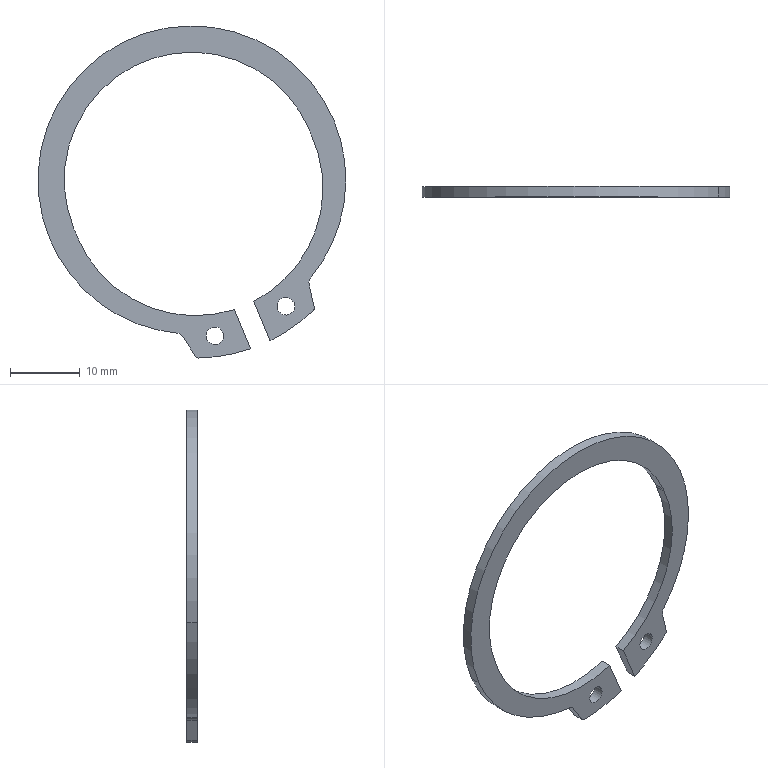Component | SolidWorks | BearingHousingAssembly-1_40ShaftRetainingRing-1 | 1 solid | 25 faces | box 44 x 1.5 x 47.45 mm | volume 704 mm3 | cylinder 19 | plane 6 | commonest cylinder face diameters 36.5 x6 2.5 x4 44 x3 2 x2 48.6 x2 1 x2
STEP:
#1=COLOUR_RGB('',0.7922,0.8196,0.9333);
#2=FILL_AREA_STYLE_COLOUR('',#1);
#3=FILL_AREA_STYLE('',(#2));
#4=SURFACE_STYLE_FILL_AREA(#3);
#5=SURFACE_SIDE_STYLE('',(#4));
#6=SURFACE_STYLE_USAGE(.BOTH.,#5);
#7=PRESENTATION_STYLE_ASSIGNMENT((#6));
#8=CARTESIAN_POINT('',(-0.8586,9.341,0.039));
#9=VERTEX_POINT('',#8);
#10=CARTESIAN_POINT('',(-0.8495,9.341,0.01611));
#11=VERTEX_POINT('',#10);
#12=CARTESIAN_POINT('',(-1.522,9.341,-0.2362));
#13=DIRECTION('',(0.,1.,0.));
#14=DIRECTION('',(-0.9237,0.,-0.383));
#15=AXIS2_PLACEMENT_3D('',#12,#13,#14);
#16=CIRCLE('',#15,0.7185);
#17=EDGE_CURVE('',#9,#11,#16,.T.);
#18=ORIENTED_EDGE('',*,*,#17,.F.);
#19=CARTESIAN_POINT('',(-0.8586,9.4,0.039));
#20=VERTEX_POINT('',#19);
#21=CARTESIAN_POINT('',(-0.8586,9.341,0.039));
#22=DIRECTION('',(0.,1.,0.));
#23=VECTOR('',#22,39.37);
#24=LINE('',#21,#23);
#25=EDGE_CURVE('',#9,#20,#24,.T.);
#26=ORIENTED_EDGE('',*,*,#25,.T.);
#27=CARTESIAN_POINT('',(-0.8495,9.4,0.01611));
#28=VERTEX_POINT('',#27);
#29=CARTESIAN_POINT('',(-1.522,9.4,-0.2362));
#30=DIRECTION('',(0.,1.,0.));
#31=DIRECTION('',(-0.9237,0.,-0.383));
#32=AXIS2_PLACEMENT_3D('',#29,#30,#31);
#33=CIRCLE('',#32,0.7185);
#34=EDGE_CURVE('',#20,#28,#33,.T.);
#35=ORIENTED_EDGE('',*,*,#34,.T.);
#36=CARTESIAN_POINT('',(-0.8495,9.371,0.01611));
#37=DIRECTION('',(0.,1.,0.));
#38=VECTOR('',#37,39.37);
#39=LINE('',#36,#38);
#40=EDGE_CURVE('',#11,#28,#39,.T.);
#41=ORIENTED_EDGE('',*,*,#40,.F.);
#42=EDGE_LOOP('',(#18,#26,#35,#41));
#43=FACE_OUTER_BOUND('',#42,.T.);
#44=CARTESIAN_POINT('',(-1.522,9.341,-0.2362));
#45=DIRECTION('',(0.,1.,0.));
#46=DIRECTION('',(-0.9237,0.,-0.383));
#47=AXIS2_PLACEMENT_3D('',#44,#45,#46);
#48=CYLINDRICAL_SURFACE('',#47,0.7185);
#49=ADVANCED_FACE('',(#43),#48,.F.);
#50=ORIENTED_EDGE('',*,*,#25,.F.);
#51=CARTESIAN_POINT('',(-2.186,9.341,-0.5114));
#52=VERTEX_POINT('',#51);
#53=CARTESIAN_POINT('',(-1.522,9.341,-0.2362));
#54=DIRECTION('',(0.,1.,0.));
#55=DIRECTION('',(-0.9237,0.,-0.383));
#56=AXIS2_PLACEMENT_3D('',#53,#54,#55);
#57=CIRCLE('',#56,0.7185);
#58=EDGE_CURVE('',#52,#9,#57,.T.);
#59=ORIENTED_EDGE('',*,*,#58,.F.);
#60=CARTESIAN_POINT('',(-2.186,9.4,-0.5114));
#61=VERTEX_POINT('',#60);
#62=CARTESIAN_POINT('',(-2.186,9.341,-0.5114));
#63=DIRECTION('',(0.,1.,0.));
#64=VECTOR('',#63,39.37);
#65=LINE('',#62,#64);
#66=EDGE_CURVE('',#52,#61,#65,.T.);
#67=ORIENTED_EDGE('',*,*,#66,.T.);
#68=CARTESIAN_POINT('',(-1.522,9.4,-0.2362));
#69=DIRECTION('',(0.,1.,0.));
#70=DIRECTION('',(-0.9237,0.,-0.383));
#71=AXIS2_PLACEMENT_3D('',#68,#69,#70);
#72=CIRCLE('',#71,0.7185);
#73=EDGE_CURVE('',#61,#20,#72,.T.);
#74=ORIENTED_EDGE('',*,*,#73,.T.);
#75=EDGE_LOOP('',(#50,#59,#67,#74));
#76=FACE_OUTER_BOUND('',#75,.T.);
#77=CARTESIAN_POINT('',(-1.522,9.341,-0.2362));
#78=DIRECTION('',(0.,1.,0.));
#79=DIRECTION('',(-0.9237,0.,-0.383));
#80=AXIS2_PLACEMENT_3D('',#77,#78,#79);
#81=CYLINDRICAL_SURFACE('',#80,0.7185);
#82=ADVANCED_FACE('',(#76),#81,.F.);
#83=CARTESIAN_POINT('',(-2.322,9.341,-0.568));
#84=VERTEX_POINT('',#83);
#85=CARTESIAN_POINT('',(-0.7222,9.341,0.09555));
#86=VERTEX_POINT('',#85);
#87=CARTESIAN_POINT('',(-1.522,9.341,-0.2362));
#88=DIRECTION('',(0.,1.,0.));
#89=DIRECTION('',(-0.9237,0.,-0.383));
#90=AXIS2_PLACEMENT_3D('',#87,#88,#89);
#91=CIRCLE('',#90,0.8661);
#92=EDGE_CURVE('',#84,#86,#91,.T.);
#93=ORIENTED_EDGE('',*,*,#92,.T.);
#94=CARTESIAN_POINT('',(-0.7222,9.4,0.09555));
#95=VERTEX_POINT('',#94);
#96=CARTESIAN_POINT('',(-0.7222,9.341,0.09555));
#97=DIRECTION('',(0.,1.,0.));
#98=VECTOR('',#97,39.37);
#99=LINE('',#96,#98);
#100=EDGE_CURVE('',#86,#95,#99,.T.);
#101=ORIENTED_EDGE('',*,*,#100,.T.);
#102=CARTESIAN_POINT('',(-2.322,9.4,-0.568));
#103=VERTEX_POINT('',#102);
#104=CARTESIAN_POINT('',(-1.522,9.4,-0.2362));
#105=DIRECTION('',(-0.,-1.,-0.));
#106=DIRECTION('',(-0.9237,0.,-0.383));
#107=AXIS2_PLACEMENT_3D('',#104,#105,#106);
#108=CIRCLE('',#107,0.8661);
#109=EDGE_CURVE('',#95,#103,#108,.T.);
#110=ORIENTED_EDGE('',*,*,#109,.T.);
#111=CARTESIAN_POINT('',(-2.322,9.341,-0.568));
#112=DIRECTION('',(0.,1.,0.));
#113=VECTOR('',#112,39.37);
#114=LINE('',#111,#113);
#115=EDGE_CURVE('',#84,#103,#114,.T.);
#116=ORIENTED_EDGE('',*,*,#115,.F.);
#117=EDGE_LOOP('',(#93,#101,#110,#116));
#118=FACE_OUTER_BOUND('',#117,.T.);
#119=CARTESIAN_POINT('',(-1.522,9.341,-0.2362));
#120=DIRECTION('',(0.,1.,0.));
#121=DIRECTION('',(-0.9237,0.,-0.383));
#122=AXIS2_PLACEMENT_3D('',#119,#120,#121);
#123=CYLINDRICAL_SURFACE('',#122,0.8661);
#124=ADVANCED_FACE('',(#118),#123,.T.);
#125=CARTESIAN_POINT('',(-1.603,9.341,-1.099));
#126=VERTEX_POINT('',#125);
#127=CARTESIAN_POINT('',(-1.522,9.341,-0.2362));
#128=DIRECTION('',(0.,1.,0.));
#129=DIRECTION('',(-0.9237,0.,-0.383));
#130=AXIS2_PLACEMENT_3D('',#127,#128,#129);
#131=CIRCLE('',#130,0.8661);
#132=EDGE_CURVE('',#126,#84,#131,.T.);
#133=ORIENTED_EDGE('',*,*,#132,.T.);
#134=ORIENTED_EDGE('',*,*,#115,.T.);
#135=CARTESIAN_POINT('',(-1.603,9.4,-1.099));
#136=VERTEX_POINT('',#135);
#137=CARTESIAN_POINT('',(-1.522,9.4,-0.2362));
#138=DIRECTION('',(-0.,-1.,-0.));
#139=DIRECTION('',(-0.9237,0.,-0.383));
#140=AXIS2_PLACEMENT_3D('',#137,#138,#139);
#141=CIRCLE('',#140,0.8661);
#142=EDGE_CURVE('',#103,#136,#141,.T.);
#143=ORIENTED_EDGE('',*,*,#142,.T.);
#144=CARTESIAN_POINT('',(-1.603,9.341,-1.099));
#145=DIRECTION('',(-0.,-1.,-0.));
#146=VECTOR('',#145,39.37);
#147=LINE('',#144,#146);
#148=EDGE_CURVE('',#136,#126,#147,.T.);
#149=ORIENTED_EDGE('',*,*,#148,.T.);
#150=EDGE_LOOP('',(#133,#134,#143,#149));
#151=FACE_OUTER_BOUND('',#150,.T.);
#152=CARTESIAN_POINT('',(-1.522,9.341,-0.2362));
#153=DIRECTION('',(0.,1.,0.));
#154=DIRECTION('',(-0.9237,0.,-0.383));
#155=AXIS2_PLACEMENT_3D('',#152,#153,#154);
#156=CYLINDRICAL_SURFACE('',#155,0.8661);
#157=ADVANCED_FACE('',(#151),#156,.T.);
#158=CARTESIAN_POINT('',(-2.167,9.341,-0.5569));
#159=VERTEX_POINT('',#158);
#160=CARTESIAN_POINT('',(-2.176,9.341,-0.534));
#161=VERTEX_POINT('',#160);
#162=CARTESIAN_POINT('',(-1.503,9.341,-0.2817));
#163=DIRECTION('',(0.,1.,0.));
#164=DIRECTION('',(-0.9237,0.,-0.383));
#165=AXIS2_PLACEMENT_3D('',#162,#163,#164);
#166=CIRCLE('',#165,0.7185);
#167=EDGE_CURVE('',#159,#161,#166,.T.);
#168=ORIENTED_EDGE('',*,*,#167,.F.);
#169=CARTESIAN_POINT('',(-2.167,9.4,-0.5569));
#170=VERTEX_POINT('',#169);
#171=CARTESIAN_POINT('',(-2.167,9.341,-0.5569));
#172=DIRECTION('',(0.,1.,0.));
#173=VECTOR('',#172,39.37);
#174=LINE('',#171,#173);
#175=EDGE_CURVE('',#159,#170,#174,.T.);
#176=ORIENTED_EDGE('',*,*,#175,.T.);
#177=CARTESIAN_POINT('',(-2.176,9.4,-0.534));
#178=VERTEX_POINT('',#177);
#179=CARTESIAN_POINT('',(-1.503,9.4,-0.2817));
#180=DIRECTION('',(0.,1.,0.));
#181=DIRECTION('',(-0.9237,0.,-0.383));
#182=AXIS2_PLACEMENT_3D('',#179,#180,#181);
#183=CIRCLE('',#182,0.7185);
#184=EDGE_CURVE('',#170,#178,#183,.T.);
#185=ORIENTED_EDGE('',*,*,#184,.T.);
#186=CARTESIAN_POINT('',(-2.176,9.371,-0.534));
#187=DIRECTION('',(-0.,-1.,-0.));
#188=VECTOR('',#187,39.37);
#189=LINE('',#186,#188);
#190=EDGE_CURVE('',#178,#161,#189,.T.);
#191=ORIENTED_EDGE('',*,*,#190,.T.);
#192=EDGE_LOOP('',(#168,#176,#185,#191));
#193=FACE_OUTER_BOUND('',#192,.T.);
#194=CARTESIAN_POINT('',(-1.503,9.341,-0.2817));
#195=DIRECTION('',(0.,1.,0.));
#196=DIRECTION('',(-0.9237,0.,-0.383));
#197=AXIS2_PLACEMENT_3D('',#194,#195,#196);
#198=CYLINDRICAL_SURFACE('',#197,0.7185);
#199=ADVANCED_FACE('',(#193),#198,.F.);
#200=CARTESIAN_POINT('',(-0.9476,9.341,-0.9282));
#201=VERTEX_POINT('',#200);
#202=CARTESIAN_POINT('',(-1.039,9.341,-0.9659));
#203=VERTEX_POINT('',#202);
#204=CARTESIAN_POINT('',(-0.9931,9.341,-0.9471));
#205=DIRECTION('',(0.,1.,0.));
#206=DIRECTION('',(-0.9237,0.,-0.383));
#207=AXIS2_PLACEMENT_3D('',#204,#205,#206);
#208=CIRCLE('',#207,0.04921);
#209=EDGE_CURVE('',#201,#203,#208,.T.);
#210=ORIENTED_EDGE('',*,*,#209,.F.);
#211=CARTESIAN_POINT('',(-0.9476,9.4,-0.9282));
#212=VERTEX_POINT('',#211);
#213=CARTESIAN_POINT('',(-0.9476,9.341,-0.9282));
#214=DIRECTION('',(0.,1.,0.));
#215=VECTOR('',#214,39.37);
#216=LINE('',#213,#215);
#217=EDGE_CURVE('',#201,#212,#216,.T.);
#218=ORIENTED_EDGE('',*,*,#217,.T.);
#219=CARTESIAN_POINT('',(-1.039,9.4,-0.9659));
#220=VERTEX_POINT('',#219);
#221=CARTESIAN_POINT('',(-0.9931,9.4,-0.9471));
#222=DIRECTION('',(0.,1.,0.));
#223=DIRECTION('',(-0.9237,0.,-0.383));
#224=AXIS2_PLACEMENT_3D('',#221,#222,#223);
#225=CIRCLE('',#224,0.04921);
#226=EDGE_CURVE('',#212,#220,#225,.T.);
#227=ORIENTED_EDGE('',*,*,#226,.T.);
#228=CARTESIAN_POINT('',(-1.039,9.341,-0.9659));
#229=DIRECTION('',(0.,1.,0.));
#230=VECTOR('',#229,39.37);
#231=LINE('',#228,#230);
#232=EDGE_CURVE('',#203,#220,#231,.T.);
#233=ORIENTED_EDGE('',*,*,#232,.F.);
#234=EDGE_LOOP('',(#210,#218,#227,#233));
#235=FACE_OUTER_BOUND('',#234,.T.);
#236=CARTESIAN_POINT('',(-0.9931,9.341,-0.9471));
#237=DIRECTION('',(0.,1.,0.));
#238=DIRECTION('',(-0.9237,0.,-0.383));
#239=AXIS2_PLACEMENT_3D('',#236,#237,#238);
#240=CYLINDRICAL_SURFACE('',#239,0.04921);
#241=ADVANCED_FACE('',(#235),#240,.F.);
#242=CARTESIAN_POINT('',(-1.348,9.341,-1.094));
#243=VERTEX_POINT('',#242);
#244=CARTESIAN_POINT('',(-1.439,9.341,-1.132));
#245=VERTEX_POINT('',#244);
#246=CARTESIAN_POINT('',(-1.393,9.341,-1.113));
#247=DIRECTION('',(0.,1.,0.));
#248=DIRECTION('',(-0.9237,0.,-0.383));
#249=AXIS2_PLACEMENT_3D('',#246,#247,#248);
#250=CIRCLE('',#249,0.04921);
#251=EDGE_CURVE('',#243,#245,#250,.T.);
#252=ORIENTED_EDGE('',*,*,#251,.F.);
#253=CARTESIAN_POINT('',(-1.348,9.4,-1.094));
#254=VERTEX_POINT('',#253);
#255=CARTESIAN_POINT('',(-1.348,9.341,-1.094));
#256=DIRECTION('',(0.,1.,0.));
#257=VECTOR('',#256,39.37);
#258=LINE('',#255,#257);
#259=EDGE_CURVE('',#243,#254,#258,.T.);
#260=ORIENTED_EDGE('',*,*,#259,.T.);
#261=CARTESIAN_POINT('',(-1.439,9.4,-1.132));
#262=VERTEX_POINT('',#261);
#263=CARTESIAN_POINT('',(-1.393,9.4,-1.113));
#264=DIRECTION('',(0.,1.,0.));
#265=DIRECTION('',(-0.9237,0.,-0.383));
#266=AXIS2_PLACEMENT_3D('',#263,#264,#265);
#267=CIRCLE('',#266,0.04921);
#268=EDGE_CURVE('',#254,#262,#267,.T.);
#269=ORIENTED_EDGE('',*,*,#268,.T.);
#270=CARTESIAN_POINT('',(-1.439,9.341,-1.132));
#271=DIRECTION('',(0.,1.,0.));
#272=VECTOR('',#271,39.37);
#273=LINE('',#270,#272);
#274=EDGE_CURVE('',#245,#262,#273,.T.);
#275=ORIENTED_EDGE('',*,*,#274,.F.);
#276=EDGE_LOOP('',(#252,#260,#269,#275));
#277=FACE_OUTER_BOUND('',#276,.T.);
#278=CARTESIAN_POINT('',(-1.393,9.341,-1.113));
#279=DIRECTION('',(0.,1.,0.));
#280=DIRECTION('',(-0.9237,0.,-0.383));
#281=AXIS2_PLACEMENT_3D('',#278,#279,#280);
#282=CYLINDRICAL_SURFACE('',#281,0.04921);
#283=ADVANCED_FACE('',(#277),#282,.F.);
#284=CARTESIAN_POINT('',(-0.9931,9.341,-0.9471));
#285=DIRECTION('',(0.,1.,0.));
#286=DIRECTION('',(-0.9237,0.,-0.383));
#287=AXIS2_PLACEMENT_3D('',#284,#285,#286);
#288=CIRCLE('',#287,0.04921);
#289=EDGE_CURVE('',#203,#201,#288,.T.);
#290=ORIENTED_EDGE('',*,*,#289,.T.);
#291=ORIENTED_EDGE('',*,*,#209,.T.);
#292=EDGE_LOOP('',(#290,#291));
#293=FACE_BOUND('',#292,.T.);
#294=CARTESIAN_POINT('',(-1.393,9.341,-1.113));
#295=DIRECTION('',(0.,1.,0.));
#296=DIRECTION('',(-0.9237,0.,-0.383));
#297=AXIS2_PLACEMENT_3D('',#294,#295,#296);
#298=CIRCLE('',#297,0.04921);
#299=EDGE_CURVE('',#245,#243,#298,.T.);
#300=ORIENTED_EDGE('',*,*,#299,.T.);
#301=ORIENTED_EDGE('',*,*,#251,.T.);
#302=EDGE_LOOP('',(#300,#301));
#303=FACE_BOUND('',#302,.T.);
#304=CARTESIAN_POINT('',(-1.284,9.341,-0.9658));
#305=VERTEX_POINT('',#304);
#306=CARTESIAN_POINT('',(-1.503,9.341,-0.2817));
#307=DIRECTION('',(0.,1.,0.));
#308=DIRECTION('',(-0.9237,0.,-0.383));
#309=AXIS2_PLACEMENT_3D('',#306,#307,#308);
#310=CIRCLE('',#309,0.7185);
#311=EDGE_CURVE('',#305,#159,#310,.T.);
#312=ORIENTED_EDGE('',*,*,#311,.T.);
#313=ORIENTED_EDGE('',*,*,#167,.T.);
#314=CARTESIAN_POINT('',(-1.522,9.341,-0.2362));
#315=DIRECTION('',(0.,1.,0.));
#316=DIRECTION('',(-0.9237,0.,-0.383));
#317=AXIS2_PLACEMENT_3D('',#314,#315,#316);
#318=CIRCLE('',#317,0.7185);
#319=EDGE_CURVE('',#161,#52,#318,.T.);
#320=ORIENTED_EDGE('',*,*,#319,.T.);
#321=ORIENTED_EDGE('',*,*,#58,.T.);
#322=ORIENTED_EDGE('',*,*,#17,.T.);
#323=CARTESIAN_POINT('',(-1.175,9.341,-0.9205));
#324=VERTEX_POINT('',#323);
#325=CARTESIAN_POINT('',(-1.503,9.341,-0.2817));
#326=DIRECTION('',(0.,1.,0.));
#327=DIRECTION('',(-0.9237,0.,-0.383));
#328=AXIS2_PLACEMENT_3D('',#325,#326,#327);
#329=CIRCLE('',#328,0.7185);
#330=EDGE_CURVE('',#11,#324,#329,.T.);
#331=ORIENTED_EDGE('',*,*,#330,.T.);
#332=CARTESIAN_POINT('',(-1.083,9.341,-1.141));
#333=VERTEX_POINT('',#332);
#334=CARTESIAN_POINT('',(-1.175,9.341,-0.9205));
#335=DIRECTION('',(-0.383,0.,0.9237));
#336=VECTOR('',#335,39.37);
#337=LINE('',#334,#336);
#338=EDGE_CURVE('',#333,#324,#337,.T.);
#339=ORIENTED_EDGE('',*,*,#338,.F.);
#340=CARTESIAN_POINT('',(-0.8395,9.341,-0.9705));
#341=VERTEX_POINT('',#340);
#342=CARTESIAN_POINT('',(-1.503,9.341,-0.2817));
#343=DIRECTION('',(0.,1.,0.));
#344=DIRECTION('',(-0.9237,0.,-0.383));
#345=AXIS2_PLACEMENT_3D('',#342,#343,#344);
#346=CIRCLE('',#345,0.9567);
#347=EDGE_CURVE('',#341,#333,#346,.T.);
#348=ORIENTED_EDGE('',*,*,#347,.F.);
#349=CARTESIAN_POINT('',(-0.8339,9.341,-0.952));
#350=VERTEX_POINT('',#349);
#351=CARTESIAN_POINT('',(-0.8531,9.341,-0.9563));
#352=DIRECTION('',(-0.,-1.,-0.));
#353=DIRECTION('',(-0.9237,0.,-0.383));
#354=AXIS2_PLACEMENT_3D('',#351,#352,#353);
#355=CIRCLE('',#354,0.01969);
#356=EDGE_CURVE('',#341,#350,#355,.T.);
#357=ORIENTED_EDGE('',*,*,#356,.T.);
#358=CARTESIAN_POINT('',(-0.8628,9.341,-0.8217));
#359=VERTEX_POINT('',#358);
#360=CARTESIAN_POINT('',(-0.8671,9.341,-0.8027));
#361=DIRECTION('',(0.2168,-0.,-0.9762));
#362=VECTOR('',#361,39.37);
#363=LINE('',#360,#362);
#364=EDGE_CURVE('',#359,#350,#363,.T.);
#365=ORIENTED_EDGE('',*,*,#364,.F.);
#366=CARTESIAN_POINT('',(-0.8547,9.341,-0.7881));
#367=VERTEX_POINT('',#366);
#368=CARTESIAN_POINT('',(-0.8244,9.341,-0.8132));
#369=DIRECTION('',(0.,1.,0.));
#370=DIRECTION('',(-0.9237,0.,-0.383));
#371=AXIS2_PLACEMENT_3D('',#368,#369,#370);
#372=CIRCLE('',#371,0.03937);
#373=EDGE_CURVE('',#359,#367,#372,.T.);
#374=ORIENTED_EDGE('',*,*,#373,.T.);
#375=CARTESIAN_POINT('',(-1.522,9.341,-0.2362));
#376=DIRECTION('',(0.,1.,0.));
#377=DIRECTION('',(-0.9237,0.,-0.383));
#378=AXIS2_PLACEMENT_3D('',#375,#376,#377);
#379=CIRCLE('',#378,0.8661);
#380=EDGE_CURVE('',#86,#367,#379,.T.);
#381=ORIENTED_EDGE('',*,*,#380,.F.);
#382=ORIENTED_EDGE('',*,*,#92,.F.);
#383=ORIENTED_EDGE('',*,*,#132,.F.);
#384=CARTESIAN_POINT('',(-1.574,9.341,-1.117));
#385=VERTEX_POINT('',#384);
#386=CARTESIAN_POINT('',(-1.607,9.341,-1.138));
#387=DIRECTION('',(0.,1.,0.));
#388=DIRECTION('',(-0.9237,0.,-0.383));
#389=AXIS2_PLACEMENT_3D('',#386,#387,#388);
#390=CIRCLE('',#389,0.03937);
#391=EDGE_CURVE('',#126,#385,#390,.T.);
#392=ORIENTED_EDGE('',*,*,#391,.T.);
#393=CARTESIAN_POINT('',(-1.502,9.341,-1.229));
#394=VERTEX_POINT('',#393);
#395=CARTESIAN_POINT('',(-1.584,9.341,-1.1));
#396=DIRECTION('',(-0.5376,0.,0.8432));
#397=VECTOR('',#396,39.37);
#398=LINE('',#395,#397);
#399=EDGE_CURVE('',#394,#385,#398,.T.);
#400=ORIENTED_EDGE('',*,*,#399,.F.);
#401=CARTESIAN_POINT('',(-1.485,9.341,-1.238));
#402=VERTEX_POINT('',#401);
#403=CARTESIAN_POINT('',(-1.486,9.341,-1.219));
#404=DIRECTION('',(-0.,-1.,-0.));
#405=DIRECTION('',(-0.9237,0.,-0.383));
#406=AXIS2_PLACEMENT_3D('',#403,#404,#405);
#407=CIRCLE('',#406,0.01969);
#408=EDGE_CURVE('',#394,#402,#407,.T.);
#409=ORIENTED_EDGE('',*,*,#408,.T.);
#410=CARTESIAN_POINT('',(-1.192,9.341,-1.186));
#411=VERTEX_POINT('',#410);
#412=CARTESIAN_POINT('',(-1.503,9.341,-0.2817));
#413=DIRECTION('',(0.,1.,0.));
#414=DIRECTION('',(-0.9237,0.,-0.383));
#415=AXIS2_PLACEMENT_3D('',#412,#413,#414);
#416=CIRCLE('',#415,0.9567);
#417=EDGE_CURVE('',#411,#402,#416,.T.);
#418=ORIENTED_EDGE('',*,*,#417,.F.);
#419=CARTESIAN_POINT('',(-1.284,9.341,-0.9658));
#420=DIRECTION('',(0.383,-0.,-0.9237));
#421=VECTOR('',#420,39.37);
#422=LINE('',#419,#421);
#423=EDGE_CURVE('',#305,#411,#422,.T.);
#424=ORIENTED_EDGE('',*,*,#423,.F.);
#425=EDGE_LOOP('',(#312,#313,#320,#321,#322,#331,#339,#348,#357,#365,#374,#381,#382,#383,#392,#400,#409,#418,#424));
#426=FACE_OUTER_BOUND('',#425,.T.);
#427=CARTESIAN_POINT('',(-1.503,9.341,-0.2817));
#428=DIRECTION('',(-0.,-1.,-0.));
#429=DIRECTION('',(0.9237,-0.,0.383));
#430=AXIS2_PLACEMENT_3D('',#427,#428,#429);
#431=PLANE('',#430);
#432=ADVANCED_FACE('',(#293,#303,#426),#431,.T.);
#433=ORIENTED_EDGE('',*,*,#330,.F.);
#434=ORIENTED_EDGE('',*,*,#40,.T.);
#435=CARTESIAN_POINT('',(-1.175,9.4,-0.9205));
#436=VERTEX_POINT('',#435);
#437=CARTESIAN_POINT('',(-1.503,9.4,-0.2817));
#438=DIRECTION('',(0.,1.,0.));
#439=DIRECTION('',(-0.9237,0.,-0.383));
#440=AXIS2_PLACEMENT_3D('',#437,#438,#439);
#441=CIRCLE('',#440,0.7185);
#442=EDGE_CURVE('',#28,#436,#441,.T.);
#443=ORIENTED_EDGE('',*,*,#442,.T.);
#444=CARTESIAN_POINT('',(-1.175,9.341,-0.9205));
#445=DIRECTION('',(0.,1.,0.));
#446=VECTOR('',#445,39.37);
#447=LINE('',#444,#446);
#448=EDGE_CURVE('',#324,#436,#447,.T.);
#449=ORIENTED_EDGE('',*,*,#448,.F.);
#450=EDGE_LOOP('',(#433,#434,#443,#449));
#451=FACE_OUTER_BOUND('',#450,.T.);
#452=CARTESIAN_POINT('',(-1.503,9.341,-0.2817));
#453=DIRECTION('',(0.,1.,0.));
#454=DIRECTION('',(-0.9237,0.,-0.383));
#455=AXIS2_PLACEMENT_3D('',#452,#453,#454);
#456=CYLINDRICAL_SURFACE('',#455,0.7185);
#457=ADVANCED_FACE('',(#451),#456,.F.);
#458=CARTESIAN_POINT('',(-1.393,9.4,-1.113));
#459=DIRECTION('',(0.,1.,0.));
#460=DIRECTION('',(-0.9237,0.,-0.383));
#461=AXIS2_PLACEMENT_3D('',#458,#459,#460);
#462=CIRCLE('',#461,0.04921);
#463=EDGE_CURVE('',#262,#254,#462,.T.);
#464=ORIENTED_EDGE('',*,*,#463,.F.);
#465=ORIENTED_EDGE('',*,*,#268,.F.);
#466=EDGE_LOOP('',(#464,#465));
#467=FACE_BOUND('',#466,.T.);
#468=CARTESIAN_POINT('',(-0.9931,9.4,-0.9471));
#469=DIRECTION('',(0.,1.,0.));
#470=DIRECTION('',(-0.9237,0.,-0.383));
#471=AXIS2_PLACEMENT_3D('',#468,#469,#470);
#472=CIRCLE('',#471,0.04921);
#473=EDGE_CURVE('',#220,#212,#472,.T.);
#474=ORIENTED_EDGE('',*,*,#473,.F.);
#475=ORIENTED_EDGE('',*,*,#226,.F.);
#476=EDGE_LOOP('',(#474,#475));
#477=FACE_BOUND('',#476,.T.);
#478=CARTESIAN_POINT('',(-1.522,9.4,-0.2362));
#479=DIRECTION('',(0.,1.,0.));
#480=DIRECTION('',(-0.9237,0.,-0.383));
#481=AXIS2_PLACEMENT_3D('',#478,#479,#480);
#482=CIRCLE('',#481,0.7185);
#483=EDGE_CURVE('',#178,#61,#482,.T.);
#484=ORIENTED_EDGE('',*,*,#483,.F.);
#485=ORIENTED_EDGE('',*,*,#184,.F.);
#486=CARTESIAN_POINT('',(-1.284,9.4,-0.9658));
#487=VERTEX_POINT('',#486);
#488=CARTESIAN_POINT('',(-1.503,9.4,-0.2817));
#489=DIRECTION('',(0.,1.,0.));
#490=DIRECTION('',(-0.9237,0.,-0.383));
#491=AXIS2_PLACEMENT_3D('',#488,#489,#490);
#492=CIRCLE('',#491,0.7185);
#493=EDGE_CURVE('',#487,#170,#492,.T.);
#494=ORIENTED_EDGE('',*,*,#493,.F.);
#495=CARTESIAN_POINT('',(-1.192,9.4,-1.186));
#496=VERTEX_POINT('',#495);
#497=CARTESIAN_POINT('',(-1.558,9.4,-0.3043));
#498=DIRECTION('',(-0.383,0.,0.9237));
#499=VECTOR('',#498,39.37);
#500=LINE('',#497,#499);
#501=EDGE_CURVE('',#496,#487,#500,.T.);
#502=ORIENTED_EDGE('',*,*,#501,.F.);
#503=CARTESIAN_POINT('',(-1.485,9.4,-1.238));
#504=VERTEX_POINT('',#503);
#505=CARTESIAN_POINT('',(-1.503,9.4,-0.2817));
#506=DIRECTION('',(-0.,-1.,-0.));
#507=DIRECTION('',(-0.9237,0.,-0.383));
#508=AXIS2_PLACEMENT_3D('',#505,#506,#507);
#509=CIRCLE('',#508,0.9567);
#510=EDGE_CURVE('',#504,#496,#509,.T.);
#511=ORIENTED_EDGE('',*,*,#510,.F.);
#512=CARTESIAN_POINT('',(-1.502,9.4,-1.229));
#513=VERTEX_POINT('',#512);
#514=CARTESIAN_POINT('',(-1.486,9.4,-1.219));
#515=DIRECTION('',(-0.,-1.,-0.));
#516=DIRECTION('',(-0.9237,0.,-0.383));
#517=AXIS2_PLACEMENT_3D('',#514,#515,#516);
#518=CIRCLE('',#517,0.01969);
#519=EDGE_CURVE('',#513,#504,#518,.T.);
#520=ORIENTED_EDGE('',*,*,#519,.F.);
#521=CARTESIAN_POINT('',(-1.574,9.4,-1.117));
#522=VERTEX_POINT('',#521);
#523=CARTESIAN_POINT('',(-1.574,9.4,-1.117));
#524=DIRECTION('',(0.5376,-0.,-0.8432));
#525=VECTOR('',#524,39.37);
#526=LINE('',#523,#525);
#527=EDGE_CURVE('',#522,#513,#526,.T.);
#528=ORIENTED_EDGE('',*,*,#527,.F.);
#529=CARTESIAN_POINT('',(-1.607,9.4,-1.138));
#530=DIRECTION('',(0.,1.,0.));
#531=DIRECTION('',(-0.9237,0.,-0.383));
#532=AXIS2_PLACEMENT_3D('',#529,#530,#531);
#533=CIRCLE('',#532,0.03937);
#534=EDGE_CURVE('',#136,#522,#533,.T.);
#535=ORIENTED_EDGE('',*,*,#534,.F.);
#536=ORIENTED_EDGE('',*,*,#142,.F.);
#537=ORIENTED_EDGE('',*,*,#109,.F.);
#538=CARTESIAN_POINT('',(-0.8547,9.4,-0.7881));
#539=VERTEX_POINT('',#538);
#540=CARTESIAN_POINT('',(-1.522,9.4,-0.2362));
#541=DIRECTION('',(-0.,-1.,-0.));
#542=DIRECTION('',(-0.9237,0.,-0.383));
#543=AXIS2_PLACEMENT_3D('',#540,#541,#542);
#544=CIRCLE('',#543,0.8661);
#545=EDGE_CURVE('',#539,#95,#544,.T.);
#546=ORIENTED_EDGE('',*,*,#545,.F.);
#547=CARTESIAN_POINT('',(-0.8628,9.4,-0.8217));
#548=VERTEX_POINT('',#547);
#549=CARTESIAN_POINT('',(-0.8244,9.4,-0.8132));
#550=DIRECTION('',(0.,1.,0.));
#551=DIRECTION('',(-0.9237,0.,-0.383));
#552=AXIS2_PLACEMENT_3D('',#549,#550,#551);
#553=CIRCLE('',#552,0.03937);
#554=EDGE_CURVE('',#548,#539,#553,.T.);
#555=ORIENTED_EDGE('',*,*,#554,.F.);
#556=CARTESIAN_POINT('',(-0.8339,9.4,-0.952));
#557=VERTEX_POINT('',#556);
#558=CARTESIAN_POINT('',(-0.8339,9.4,-0.952));
#559=DIRECTION('',(-0.2168,0.,0.9762));
#560=VECTOR('',#559,39.37);
#561=LINE('',#558,#560);
#562=EDGE_CURVE('',#557,#548,#561,.T.);
#563=ORIENTED_EDGE('',*,*,#562,.F.);
#564=CARTESIAN_POINT('',(-0.8395,9.4,-0.9705));
#565=VERTEX_POINT('',#564);
#566=CARTESIAN_POINT('',(-0.8531,9.4,-0.9563));
#567=DIRECTION('',(-0.,-1.,-0.));
#568=DIRECTION('',(-0.9237,0.,-0.383));
#569=AXIS2_PLACEMENT_3D('',#566,#567,#568);
#570=CIRCLE('',#569,0.01969);
#571=EDGE_CURVE('',#565,#557,#570,.T.);
#572=ORIENTED_EDGE('',*,*,#571,.F.);
#573=CARTESIAN_POINT('',(-1.083,9.4,-1.141));
#574=VERTEX_POINT('',#573);
#575=CARTESIAN_POINT('',(-1.503,9.4,-0.2817));
#576=DIRECTION('',(-0.,-1.,-0.));
#577=DIRECTION('',(-0.9237,0.,-0.383));
#578=AXIS2_PLACEMENT_3D('',#575,#576,#577);
#579=CIRCLE('',#578,0.9567);
#580=EDGE_CURVE('',#574,#565,#579,.T.);
#581=ORIENTED_EDGE('',*,*,#580,.F.);
#582=CARTESIAN_POINT('',(-1.449,9.4,-0.2591));
#583=DIRECTION('',(0.383,-0.,-0.9237));
#584=VECTOR('',#583,39.37);
#585=LINE('',#582,#584);
#586=EDGE_CURVE('',#436,#574,#585,.T.);
#587=ORIENTED_EDGE('',*,*,#586,.F.);
#588=ORIENTED_EDGE('',*,*,#442,.F.);
#589=ORIENTED_EDGE('',*,*,#34,.F.);
#590=ORIENTED_EDGE('',*,*,#73,.F.);
#591=EDGE_LOOP('',(#484,#485,#494,#502,#511,#520,#528,#535,#536,#537,#546,#555,#563,#572,#581,#587,#588,#589,#590));
#592=FACE_OUTER_BOUND('',#591,.T.);
#593=CARTESIAN_POINT('',(-1.503,9.4,-0.2817));
#594=DIRECTION('',(-0.,-1.,-0.));
#595=DIRECTION('',(0.9237,-0.,0.383));
#596=AXIS2_PLACEMENT_3D('',#593,#594,#595);
#597=PLANE('',#596);
#598=ADVANCED_FACE('',(#467,#477,#592),#597,.F.);
#599=ORIENTED_EDGE('',*,*,#100,.F.);
#600=ORIENTED_EDGE('',*,*,#380,.T.);
#601=CARTESIAN_POINT('',(-0.8547,9.341,-0.7881));
#602=DIRECTION('',(0.,1.,0.));
#603=VECTOR('',#602,39.37);
#604=LINE('',#601,#603);
#605=EDGE_CURVE('',#367,#539,#604,.T.);
#606=ORIENTED_EDGE('',*,*,#605,.T.);
#607=ORIENTED_EDGE('',*,*,#545,.T.);
#608=EDGE_LOOP('',(#599,#600,#606,#607));
#609=FACE_OUTER_BOUND('',#608,.T.);
#610=CARTESIAN_POINT('',(-1.522,9.341,-0.2362));
#611=DIRECTION('',(0.,1.,0.));
#612=DIRECTION('',(-0.9237,0.,-0.383));
#613=AXIS2_PLACEMENT_3D('',#610,#611,#612);
#614=CYLINDRICAL_SURFACE('',#613,0.8661);
#615=ADVANCED_FACE('',(#609),#614,.T.);
#616=CARTESIAN_POINT('',(-0.8628,9.341,-0.8217));
#617=DIRECTION('',(-0.,-1.,-0.));
#618=VECTOR('',#617,39.37);
#619=LINE('',#616,#618);
#620=EDGE_CURVE('',#548,#359,#619,.T.);
#621=ORIENTED_EDGE('',*,*,#620,.F.);
#622=ORIENTED_EDGE('',*,*,#554,.T.);
#623=ORIENTED_EDGE('',*,*,#605,.F.);
#624=ORIENTED_EDGE('',*,*,#373,.F.);
#625=EDGE_LOOP('',(#621,#622,#623,#624));
#626=FACE_OUTER_BOUND('',#625,.T.);
#627=CARTESIAN_POINT('',(-0.8244,9.341,-0.8132));
#628=DIRECTION('',(0.,1.,0.));
#629=DIRECTION('',(-0.9237,0.,-0.383));
#630=AXIS2_PLACEMENT_3D('',#627,#628,#629);
#631=CYLINDRICAL_SURFACE('',#630,0.03937);
#632=ADVANCED_FACE('',(#626),#631,.F.);
#633=ORIENTED_EDGE('',*,*,#364,.T.);
#634=CARTESIAN_POINT('',(-0.8339,9.341,-0.952));
#635=DIRECTION('',(0.,1.,0.));
#636=VECTOR('',#635,39.37);
#637=LINE('',#634,#636);
#638=EDGE_CURVE('',#350,#557,#637,.T.);
#639=ORIENTED_EDGE('',*,*,#638,.T.);
#640=ORIENTED_EDGE('',*,*,#562,.T.);
#641=ORIENTED_EDGE('',*,*,#620,.T.);
#642=EDGE_LOOP('',(#633,#639,#640,#641));
#643=FACE_OUTER_BOUND('',#642,.T.);
#644=CARTESIAN_POINT('',(-0.8671,9.341,-0.8027));
#645=DIRECTION('',(0.9762,-0.,0.2168));
#646=DIRECTION('',(0.2168,-0.,-0.9762));
#647=AXIS2_PLACEMENT_3D('',#644,#645,#646);
#648=PLANE('',#647);
#649=ADVANCED_FACE('',(#643),#648,.T.);
#650=ORIENTED_EDGE('',*,*,#347,.T.);
#651=CARTESIAN_POINT('',(-1.083,9.341,-1.141));
#652=DIRECTION('',(0.,1.,0.));
#653=VECTOR('',#652,39.37);
#654=LINE('',#651,#653);
#655=EDGE_CURVE('',#333,#574,#654,.T.);
#656=ORIENTED_EDGE('',*,*,#655,.T.);
#657=ORIENTED_EDGE('',*,*,#580,.T.);
#658=CARTESIAN_POINT('',(-0.8395,9.341,-0.9705));
#659=DIRECTION('',(-0.,-1.,-0.));
#660=VECTOR('',#659,39.37);
#661=LINE('',#658,#660);
#662=EDGE_CURVE('',#565,#341,#661,.T.);
#663=ORIENTED_EDGE('',*,*,#662,.T.);
#664=EDGE_LOOP('',(#650,#656,#657,#663));
#665=FACE_OUTER_BOUND('',#664,.T.);
#666=CARTESIAN_POINT('',(-1.503,9.341,-0.2817));
#667=DIRECTION('',(0.,1.,0.));
#668=DIRECTION('',(-0.9237,0.,-0.383));
#669=AXIS2_PLACEMENT_3D('',#666,#667,#668);
#670=CYLINDRICAL_SURFACE('',#669,0.9567);
#671=ADVANCED_FACE('',(#665),#670,.T.);
#672=ORIENTED_EDGE('',*,*,#338,.T.);
#673=ORIENTED_EDGE('',*,*,#448,.T.);
#674=ORIENTED_EDGE('',*,*,#586,.T.);
#675=ORIENTED_EDGE('',*,*,#655,.F.);
#676=EDGE_LOOP('',(#672,#673,#674,#675));
#677=FACE_OUTER_BOUND('',#676,.T.);
#678=CARTESIAN_POINT('',(-1.175,9.341,-0.9205));
#679=DIRECTION('',(-0.9237,0.,-0.383));
#680=DIRECTION('',(-0.,-1.,-0.));
#681=AXIS2_PLACEMENT_3D('',#678,#679,#680);
#682=PLANE('',#681);
#683=ADVANCED_FACE('',(#677),#682,.T.);
#684=ORIENTED_EDGE('',*,*,#175,.F.);
#685=ORIENTED_EDGE('',*,*,#311,.F.);
#686=CARTESIAN_POINT('',(-1.284,9.341,-0.9658));
#687=DIRECTION('',(-0.,-1.,-0.));
#688=VECTOR('',#687,39.37);
#689=LINE('',#686,#688);
#690=EDGE_CURVE('',#487,#305,#689,.T.);
#691=ORIENTED_EDGE('',*,*,#690,.F.);
#692=ORIENTED_EDGE('',*,*,#493,.T.);
#693=EDGE_LOOP('',(#684,#685,#691,#692));
#694=FACE_OUTER_BOUND('',#693,.T.);
#695=CARTESIAN_POINT('',(-1.503,9.341,-0.2817));
#696=DIRECTION('',(0.,1.,0.));
#697=DIRECTION('',(-0.9237,0.,-0.383));
#698=AXIS2_PLACEMENT_3D('',#695,#696,#697);
#699=CYLINDRICAL_SURFACE('',#698,0.7185);
#700=ADVANCED_FACE('',(#694),#699,.F.);
#701=ORIENTED_EDGE('',*,*,#423,.T.);
#702=CARTESIAN_POINT('',(-1.192,9.341,-1.186));
#703=DIRECTION('',(0.,1.,0.));
#704=VECTOR('',#703,39.37);
#705=LINE('',#702,#704);
#706=EDGE_CURVE('',#411,#496,#705,.T.);
#707=ORIENTED_EDGE('',*,*,#706,.T.);
#708=ORIENTED_EDGE('',*,*,#501,.T.);
#709=ORIENTED_EDGE('',*,*,#690,.T.);
#710=EDGE_LOOP('',(#701,#707,#708,#709));
#711=FACE_OUTER_BOUND('',#710,.T.);
#712=CARTESIAN_POINT('',(-1.284,9.341,-0.9658));
#713=DIRECTION('',(0.9237,-0.,0.383));
#714=DIRECTION('',(0.,1.,0.));
#715=AXIS2_PLACEMENT_3D('',#712,#713,#714);
#716=PLANE('',#715);
#717=ADVANCED_FACE('',(#711),#716,.T.);
#718=ORIENTED_EDGE('',*,*,#510,.T.);
#719=ORIENTED_EDGE('',*,*,#706,.F.);
#720=ORIENTED_EDGE('',*,*,#417,.T.);
#721=CARTESIAN_POINT('',(-1.485,9.341,-1.238));
#722=DIRECTION('',(0.,1.,0.));
#723=VECTOR('',#722,39.37);
#724=LINE('',#721,#723);
#725=EDGE_CURVE('',#402,#504,#724,.T.);
#726=ORIENTED_EDGE('',*,*,#725,.T.);
#727=EDGE_LOOP('',(#718,#719,#720,#726));
#728=FACE_OUTER_BOUND('',#727,.T.);
#729=CARTESIAN_POINT('',(-1.503,9.341,-0.2817));
#730=DIRECTION('',(0.,1.,0.));
#731=DIRECTION('',(-0.9237,0.,-0.383));
#732=AXIS2_PLACEMENT_3D('',#729,#730,#731);
#733=CYLINDRICAL_SURFACE('',#732,0.9567);
#734=ADVANCED_FACE('',(#728),#733,.T.);
#735=ORIENTED_EDGE('',*,*,#527,.T.);
#736=CARTESIAN_POINT('',(-1.502,9.341,-1.229));
#737=DIRECTION('',(-0.,-1.,-0.));
#738=VECTOR('',#737,39.37);
#739=LINE('',#736,#738);
#740=EDGE_CURVE('',#513,#394,#739,.T.);
#741=ORIENTED_EDGE('',*,*,#740,.T.);
#742=ORIENTED_EDGE('',*,*,#399,.T.);
#743=CARTESIAN_POINT('',(-1.574,9.341,-1.117));
#744=DIRECTION('',(0.,1.,0.));
#745=VECTOR('',#744,39.37);
#746=LINE('',#743,#745);
#747=EDGE_CURVE('',#385,#522,#746,.T.);
#748=ORIENTED_EDGE('',*,*,#747,.T.);
#749=EDGE_LOOP('',(#735,#741,#742,#748));
#750=FACE_OUTER_BOUND('',#749,.T.);
#751=CARTESIAN_POINT('',(-1.584,9.341,-1.1));
#752=DIRECTION('',(-0.8432,0.,-0.5376));
#753=DIRECTION('',(-0.5376,0.,0.8432));
#754=AXIS2_PLACEMENT_3D('',#751,#752,#753);
#755=PLANE('',#754);
#756=ADVANCED_FACE('',(#750),#755,.T.);
#757=ORIENTED_EDGE('',*,*,#148,.F.);
#758=ORIENTED_EDGE('',*,*,#534,.T.);
#759=ORIENTED_EDGE('',*,*,#747,.F.);
#760=ORIENTED_EDGE('',*,*,#391,.F.);
#761=EDGE_LOOP('',(#757,#758,#759,#760));
#762=FACE_OUTER_BOUND('',#761,.T.);
#763=CARTESIAN_POINT('',(-1.607,9.341,-1.138));
#764=DIRECTION('',(0.,1.,0.));
#765=DIRECTION('',(-0.9237,0.,-0.383));
#766=AXIS2_PLACEMENT_3D('',#763,#764,#765);
#767=CYLINDRICAL_SURFACE('',#766,0.03937);
#768=ADVANCED_FACE('',(#762),#767,.F.);
#769=ORIENTED_EDGE('',*,*,#217,.F.);
#770=ORIENTED_EDGE('',*,*,#289,.F.);
#771=ORIENTED_EDGE('',*,*,#232,.T.);
#772=ORIENTED_EDGE('',*,*,#473,.T.);
#773=EDGE_LOOP('',(#769,#770,#771,#772));
#774=FACE_OUTER_BOUND('',#773,.T.);
#775=CARTESIAN_POINT('',(-0.9931,9.341,-0.9471));
#776=DIRECTION('',(0.,1.,0.));
#777=DIRECTION('',(-0.9237,0.,-0.383));
#778=AXIS2_PLACEMENT_3D('',#775,#776,#777);
#779=CYLINDRICAL_SURFACE('',#778,0.04921);
#780=ADVANCED_FACE('',(#774),#779,.F.);
#781=ORIENTED_EDGE('',*,*,#259,.F.);
#782=ORIENTED_EDGE('',*,*,#299,.F.);
#783=ORIENTED_EDGE('',*,*,#274,.T.);
#784=ORIENTED_EDGE('',*,*,#463,.T.);
#785=EDGE_LOOP('',(#781,#782,#783,#784));
#786=FACE_OUTER_BOUND('',#785,.T.);
#787=CARTESIAN_POINT('',(-1.393,9.341,-1.113));
#788=DIRECTION('',(0.,1.,0.));
#789=DIRECTION('',(-0.9237,0.,-0.383));
#790=AXIS2_PLACEMENT_3D('',#787,#788,#789);
#791=CYLINDRICAL_SURFACE('',#790,0.04921);
#792=ADVANCED_FACE('',(#786),#791,.F.);
#793=ORIENTED_EDGE('',*,*,#571,.T.);
#794=ORIENTED_EDGE('',*,*,#638,.F.);
#795=ORIENTED_EDGE('',*,*,#356,.F.);
#796=ORIENTED_EDGE('',*,*,#662,.F.);
#797=EDGE_LOOP('',(#793,#794,#795,#796));
#798=FACE_OUTER_BOUND('',#797,.T.);
#799=CARTESIAN_POINT('',(-0.8531,9.341,-0.9563));
#800=DIRECTION('',(0.,1.,0.));
#801=DIRECTION('',(-0.9237,0.,-0.383));
#802=AXIS2_PLACEMENT_3D('',#799,#800,#801);
#803=CYLINDRICAL_SURFACE('',#802,0.01969);
#804=ADVANCED_FACE('',(#798),#803,.T.);
#805=ORIENTED_EDGE('',*,*,#519,.T.);
#806=ORIENTED_EDGE('',*,*,#725,.F.);
#807=ORIENTED_EDGE('',*,*,#408,.F.);
#808=ORIENTED_EDGE('',*,*,#740,.F.);
#809=EDGE_LOOP('',(#805,#806,#807,#808));
#810=FACE_OUTER_BOUND('',#809,.T.);
#811=CARTESIAN_POINT('',(-1.486,9.341,-1.219));
#812=DIRECTION('',(0.,1.,0.));
#813=DIRECTION('',(-0.9237,0.,-0.383));
#814=AXIS2_PLACEMENT_3D('',#811,#812,#813);
#815=CYLINDRICAL_SURFACE('',#814,0.01969);
#816=ADVANCED_FACE('',(#810),#815,.T.);
#817=ORIENTED_EDGE('',*,*,#66,.F.);
#818=ORIENTED_EDGE('',*,*,#319,.F.);
#819=ORIENTED_EDGE('',*,*,#190,.F.);
#820=ORIENTED_EDGE('',*,*,#483,.T.);
#821=EDGE_LOOP('',(#817,#818,#819,#820));
#822=FACE_OUTER_BOUND('',#821,.T.);
#823=CARTESIAN_POINT('',(-1.522,9.341,-0.2362));
#824=DIRECTION('',(0.,1.,0.));
#825=DIRECTION('',(-0.9237,0.,-0.383));
#826=AXIS2_PLACEMENT_3D('',#823,#824,#825);
#827=CYLINDRICAL_SURFACE('',#826,0.7185);
#828=ADVANCED_FACE('',(#822),#827,.F.);
#829=CLOSED_SHELL('',(#49,#82,#124,#157,#199,#241,#283,#432,#457,#598,#615,#632,#649,#671,#683,#700,#717,#734,#756,#768,#780,#792,#804,#816,#828));
#830=MANIFOLD_SOLID_BREP('',#829);
#831=STYLED_ITEM('',(#7),#830);
#832=(LENGTH_UNIT()NAMED_UNIT(*)SI_UNIT($,.METRE.));
#833=LENGTH_MEASURE_WITH_UNIT(LENGTH_MEASURE(0.0254),#832);
#834=DIMENSIONAL_EXPONENTS(1.,0.,0.,0.,0.,0.,0.);
#835=(CONVERSION_BASED_UNIT('',#833)LENGTH_UNIT()NAMED_UNIT(#834));
#836=UNCERTAINTY_MEASURE_WITH_UNIT(LENGTH_MEASURE(0.00001),#835,'','');
#837=(NAMED_UNIT(*)PLANE_ANGLE_UNIT()SI_UNIT($,.RADIAN.));
#838=(NAMED_UNIT(*)SI_UNIT($,.STERADIAN.)SOLID_ANGLE_UNIT());
#839=(GEOMETRIC_REPRESENTATION_CONTEXT(3)GLOBAL_UNCERTAINTY_ASSIGNED_CONTEXT((#836))GLOBAL_UNIT_ASSIGNED_CONTEXT((#835,#837,#838))REPRESENTATION_CONTEXT('',''));
#840=MECHANICAL_DESIGN_GEOMETRIC_PRESENTATION_REPRESENTATION('',(#831),#839);
#841=PRESENTATION_LAYER_ASSIGNMENT('','',(#831));
#842=CARTESIAN_POINT('',(0.,0.,0.));
#843=DIRECTION('',(0.,0.,1.));
#844=DIRECTION('',(1.,0.,0.));
#845=AXIS2_PLACEMENT_3D('',#842,#843,#844);
#846=(LENGTH_UNIT()NAMED_UNIT(*)SI_UNIT($,.METRE.));
#847=LENGTH_MEASURE_WITH_UNIT(LENGTH_MEASURE(0.0254),#846);
#848=DIMENSIONAL_EXPONENTS(1.,0.,0.,0.,0.,0.,0.);
#849=(CONVERSION_BASED_UNIT('',#847)LENGTH_UNIT()NAMED_UNIT(#848));
#850=UNCERTAINTY_MEASURE_WITH_UNIT(LENGTH_MEASURE(0.00001),#849,'','');
#851=(NAMED_UNIT(*)PLANE_ANGLE_UNIT()SI_UNIT($,.RADIAN.));
#852=(NAMED_UNIT(*)SI_UNIT($,.STERADIAN.)SOLID_ANGLE_UNIT());
#853=(GEOMETRIC_REPRESENTATION_CONTEXT(3)GLOBAL_UNCERTAINTY_ASSIGNED_CONTEXT((#850))GLOBAL_UNIT_ASSIGNED_CONTEXT((#849,#851,#852))REPRESENTATION_CONTEXT('',''));
#854=ADVANCED_BREP_SHAPE_REPRESENTATION('',(#830,#845),#853);